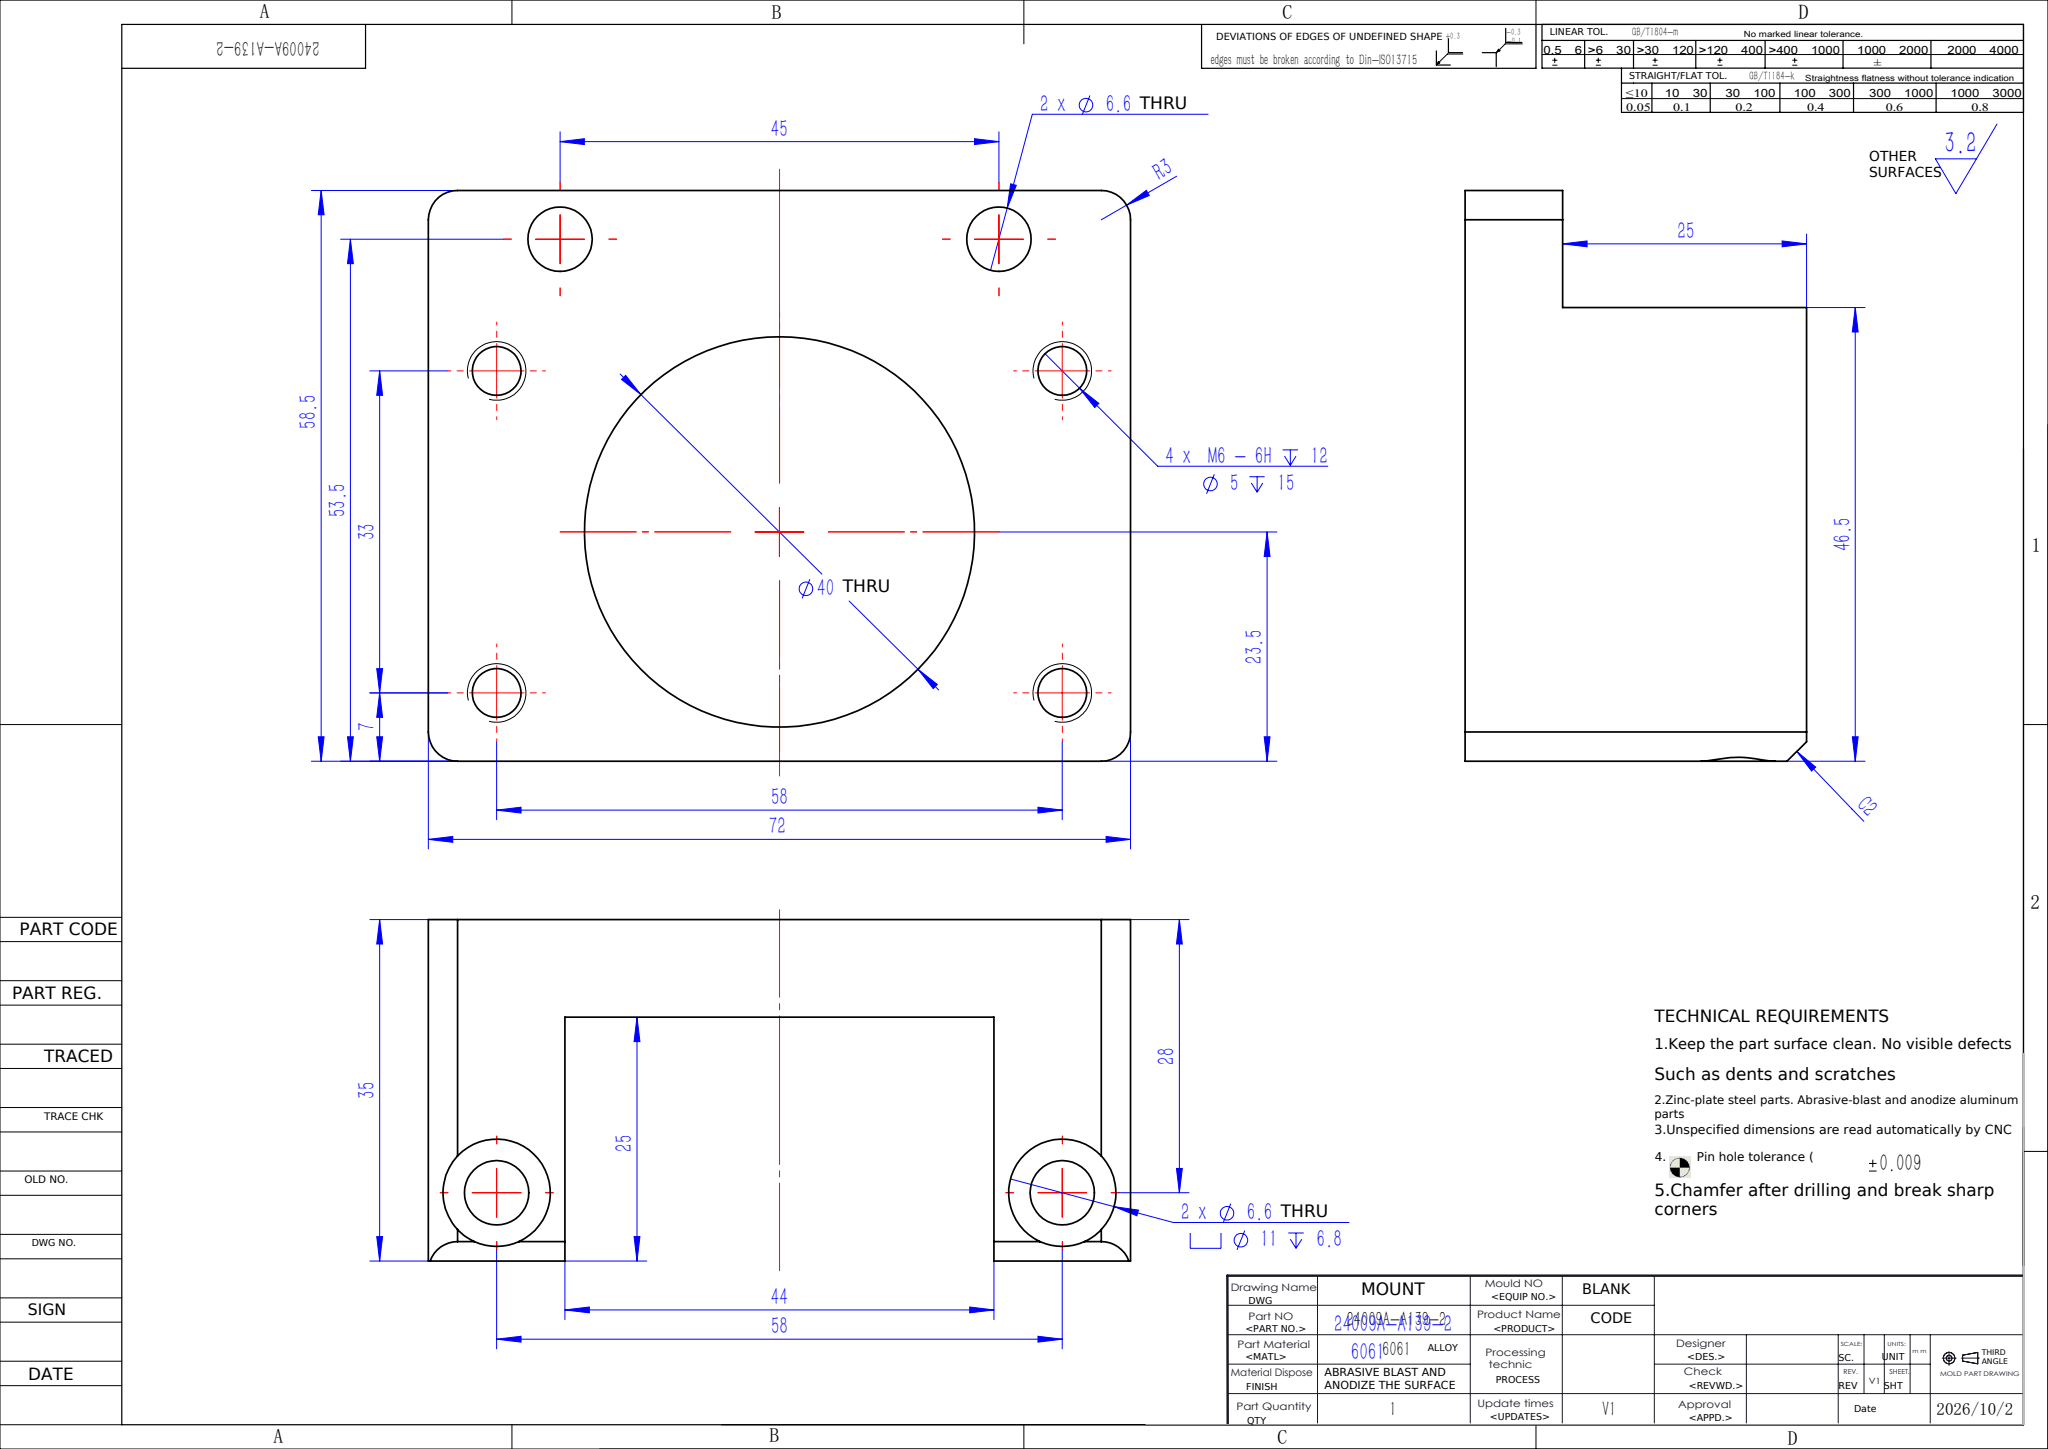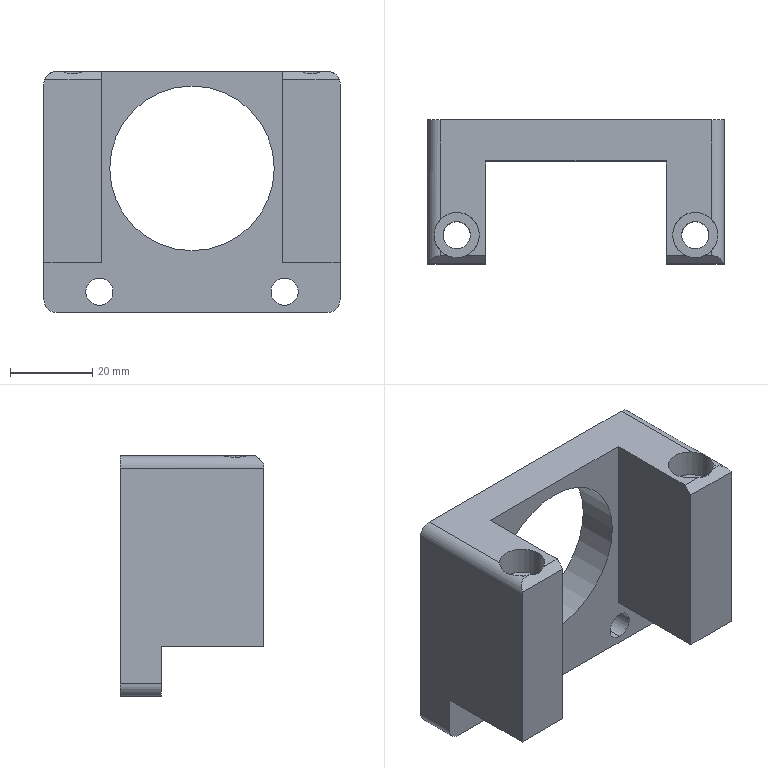Part | SolidWorks | mm | 1 solid | 52 faces | box 72 x 35 x 58.5 mm | volume 55970 mm3 | cylinder 26 | plane 18 | cone 8 | commonest cylinder face diameters 6.6 x8 5 x8 11 x4 6 x4 40 x2